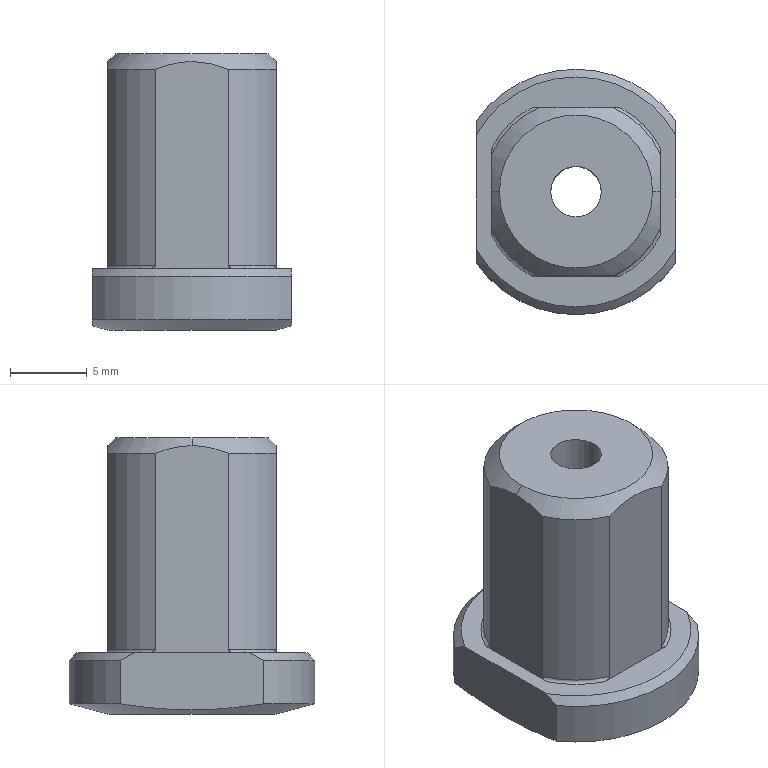Component | SolidWorks | DZ.KX.203-TC1505-30-09-01-05-18-1 | 1 solid | 27 faces | box 13 x 16 x 18 mm | volume 2023 mm3 | plane 9 | cylinder 8 | cone 6 | torus 4 | commonest cylinder face diameters 12 x4 3.3 x2 16 x2
STEP:
#1=COLOUR_RGB('',0.7922,0.8196,0.9333);
#2=FILL_AREA_STYLE_COLOUR('',#1);
#3=FILL_AREA_STYLE('',(#2));
#4=SURFACE_STYLE_FILL_AREA(#3);
#5=SURFACE_SIDE_STYLE('',(#4));
#6=SURFACE_STYLE_USAGE(.BOTH.,#5);
#7=PRESENTATION_STYLE_ASSIGNMENT((#6));
#8=CARTESIAN_POINT('',(11.53,-22.689,0.6716));
#9=VERTEX_POINT('',#8);
#10=CARTESIAN_POINT('',(11.659,-22.689,0.6716));
#11=VERTEX_POINT('',#10);
#12=CARTESIAN_POINT('',(11.594,-22.689,0.6716));
#13=DIRECTION('',(0.,0.,1.));
#14=DIRECTION('',(1.,0.,0.));
#15=AXIS2_PLACEMENT_3D('',#12,#13,#14);
#16=CIRCLE('',#15,0.06496);
#17=EDGE_CURVE('',#9,#11,#16,.T.);
#18=ORIENTED_EDGE('',*,*,#17,.F.);
#19=CARTESIAN_POINT('',(11.53,-22.689,1.38));
#20=VERTEX_POINT('',#19);
#21=CARTESIAN_POINT('',(11.53,-22.689,1.38));
#22=DIRECTION('',(0.,0.,1.));
#23=VECTOR('',#22,39.37);
#24=LINE('',#21,#23);
#25=EDGE_CURVE('',#9,#20,#24,.T.);
#26=ORIENTED_EDGE('',*,*,#25,.T.);
#27=CARTESIAN_POINT('',(11.659,-22.689,1.38));
#28=VERTEX_POINT('',#27);
#29=CARTESIAN_POINT('',(11.594,-22.689,1.38));
#30=DIRECTION('',(0.,0.,1.));
#31=DIRECTION('',(1.,0.,0.));
#32=AXIS2_PLACEMENT_3D('',#29,#30,#31);
#33=CIRCLE('',#32,0.06496);
#34=EDGE_CURVE('',#20,#28,#33,.T.);
#35=ORIENTED_EDGE('',*,*,#34,.T.);
#36=CARTESIAN_POINT('',(11.659,-22.689,1.38));
#37=DIRECTION('',(0.,0.,1.));
#38=VECTOR('',#37,39.37);
#39=LINE('',#36,#38);
#40=EDGE_CURVE('',#11,#28,#39,.T.);
#41=ORIENTED_EDGE('',*,*,#40,.F.);
#42=EDGE_LOOP('',(#18,#26,#35,#41));
#43=FACE_OUTER_BOUND('',#42,.T.);
#44=CARTESIAN_POINT('',(11.594,-22.689,1.38));
#45=DIRECTION('',(0.,0.,1.));
#46=DIRECTION('',(1.,0.,0.));
#47=AXIS2_PLACEMENT_3D('',#44,#45,#46);
#48=CYLINDRICAL_SURFACE('',#47,0.06496);
#49=ADVANCED_FACE('',(#43),#48,.F.);
#50=CARTESIAN_POINT('',(11.378,-22.689,0.6716));
#51=VERTEX_POINT('',#50);
#52=CARTESIAN_POINT('',(11.811,-22.689,0.6716));
#53=VERTEX_POINT('',#52);
#54=CARTESIAN_POINT('',(11.594,-22.689,0.6716));
#55=DIRECTION('',(-0.,-0.,-1.));
#56=DIRECTION('',(-1.,0.,0.));
#57=AXIS2_PLACEMENT_3D('',#54,#55,#56);
#58=CIRCLE('',#57,0.2165);
#59=EDGE_CURVE('',#51,#53,#58,.T.);
#60=ORIENTED_EDGE('',*,*,#59,.F.);
#61=CARTESIAN_POINT('',(11.339,-22.689,0.6822));
#62=VERTEX_POINT('',#61);
#63=CARTESIAN_POINT('',(11.28,-22.689,0.698));
#64=DIRECTION('',(-0.9659,0.,0.2588));
#65=VECTOR('',#64,39.37);
#66=LINE('',#63,#65);
#67=EDGE_CURVE('',#51,#62,#66,.T.);
#68=ORIENTED_EDGE('',*,*,#67,.T.);
#69=CARTESIAN_POINT('',(11.339,-22.506,0.698));
#70=VERTEX_POINT('',#69);
#71=CARTESIAN_POINT('',(11.339,-22.689,0.6822));
#72=CARTESIAN_POINT('',(11.339,-22.659,0.6822));
#73=CARTESIAN_POINT('',(11.339,-22.628,0.6837));
#74=CARTESIAN_POINT('',(11.339,-22.567,0.6892));
#75=CARTESIAN_POINT('',(11.339,-22.536,0.6933));
#76=CARTESIAN_POINT('',(11.339,-22.506,0.698));
#77=B_SPLINE_CURVE_WITH_KNOTS('',3,(#71,#72,#73,#74,#75,#76),.UNSPECIFIED.,.F.,.F.,(4,2,4),(0.0133,0.01565,0.018),.UNSPECIFIED.);
#78=EDGE_CURVE('',#62,#70,#77,.T.);
#79=ORIENTED_EDGE('',*,*,#78,.T.);
#80=CARTESIAN_POINT('',(11.85,-22.506,0.698));
#81=VERTEX_POINT('',#80);
#82=CARTESIAN_POINT('',(11.594,-22.689,0.698));
#83=DIRECTION('',(-0.,-0.,-1.));
#84=DIRECTION('',(-1.,0.,0.));
#85=AXIS2_PLACEMENT_3D('',#82,#83,#84);
#86=CIRCLE('',#85,0.315);
#87=EDGE_CURVE('',#70,#81,#86,.T.);
#88=ORIENTED_EDGE('',*,*,#87,.T.);
#89=CARTESIAN_POINT('',(11.85,-22.689,0.6822));
#90=VERTEX_POINT('',#89);
#91=CARTESIAN_POINT('',(11.85,-22.506,0.698));
#92=CARTESIAN_POINT('',(11.85,-22.536,0.6933));
#93=CARTESIAN_POINT('',(11.85,-22.567,0.6892));
#94=CARTESIAN_POINT('',(11.85,-22.628,0.6837));
#95=CARTESIAN_POINT('',(11.85,-22.659,0.6822));
#96=CARTESIAN_POINT('',(11.85,-22.689,0.6822));
#97=B_SPLINE_CURVE_WITH_KNOTS('',3,(#91,#92,#93,#94,#95,#96),.UNSPECIFIED.,.F.,.F.,(4,2,4),(0.02781,0.03015,0.03249),.UNSPECIFIED.);
#98=EDGE_CURVE('',#81,#90,#97,.T.);
#99=ORIENTED_EDGE('',*,*,#98,.T.);
#100=CARTESIAN_POINT('',(11.909,-22.689,0.698));
#101=DIRECTION('',(0.9659,0.,0.2588));
#102=VECTOR('',#101,39.37);
#103=LINE('',#100,#102);
#104=EDGE_CURVE('',#53,#90,#103,.T.);
#105=ORIENTED_EDGE('',*,*,#104,.F.);
#106=EDGE_LOOP('',(#60,#68,#79,#88,#99,#105));
#107=FACE_OUTER_BOUND('',#106,.T.);
#108=CARTESIAN_POINT('',(11.594,-22.689,0.698));
#109=DIRECTION('',(0.,0.,1.));
#110=DIRECTION('',(1.,0.,-0.));
#111=AXIS2_PLACEMENT_3D('',#108,#109,#110);
#112=CONICAL_SURFACE('',#111,0.315,1.309);
#113=ADVANCED_FACE('',(#107),#112,.T.);
#114=CARTESIAN_POINT('',(11.398,-22.689,1.38));
#115=VERTEX_POINT('',#114);
#116=CARTESIAN_POINT('',(11.791,-22.689,1.38));
#117=VERTEX_POINT('',#116);
#118=CARTESIAN_POINT('',(11.594,-22.689,1.38));
#119=DIRECTION('',(-0.,-0.,-1.));
#120=DIRECTION('',(-1.,0.,0.));
#121=AXIS2_PLACEMENT_3D('',#118,#119,#120);
#122=CIRCLE('',#121,0.1969);
#123=EDGE_CURVE('',#115,#117,#122,.T.);
#124=ORIENTED_EDGE('',*,*,#123,.T.);
#125=CARTESIAN_POINT('',(11.811,-22.689,1.361));
#126=VERTEX_POINT('',#125);
#127=CARTESIAN_POINT('',(11.791,-22.689,1.38));
#128=DIRECTION('',(0.7071,-0.,-0.7071));
#129=VECTOR('',#128,39.37);
#130=LINE('',#127,#129);
#131=EDGE_CURVE('',#117,#126,#130,.T.);
#132=ORIENTED_EDGE('',*,*,#131,.T.);
#133=CARTESIAN_POINT('',(11.811,-22.595,1.341));
#134=VERTEX_POINT('',#133);
#135=CARTESIAN_POINT('',(11.811,-22.595,1.341));
#136=CARTESIAN_POINT('',(11.811,-22.61,1.347));
#137=CARTESIAN_POINT('',(11.811,-22.625,1.352));
#138=CARTESIAN_POINT('',(11.811,-22.649,1.357));
#139=CARTESIAN_POINT('',(11.811,-22.657,1.358));
#140=CARTESIAN_POINT('',(11.811,-22.673,1.36));
#141=CARTESIAN_POINT('',(11.811,-22.681,1.361));
#142=CARTESIAN_POINT('',(11.811,-22.689,1.361));
#143=B_SPLINE_CURVE_WITH_KNOTS('',3,(#135,#136,#137,#138,#139,#140,#141,#142),.UNSPECIFIED.,.F.,.F.,(4,2,2,4),(0.004827,0.006044,0.006653,0.007262),.UNSPECIFIED.);
#144=EDGE_CURVE('',#134,#126,#143,.T.);
#145=ORIENTED_EDGE('',*,*,#144,.F.);
#146=CARTESIAN_POINT('',(11.689,-22.473,1.341));
#147=VERTEX_POINT('',#146);
#148=CARTESIAN_POINT('',(11.594,-22.689,1.341));
#149=DIRECTION('',(-0.,-0.,-1.));
#150=DIRECTION('',(-1.,0.,0.));
#151=AXIS2_PLACEMENT_3D('',#148,#149,#150);
#152=CIRCLE('',#151,0.2362);
#153=EDGE_CURVE('',#147,#134,#152,.T.);
#154=ORIENTED_EDGE('',*,*,#153,.F.);
#155=CARTESIAN_POINT('',(11.5,-22.473,1.341));
#156=VERTEX_POINT('',#155);
#157=CARTESIAN_POINT('',(11.5,-22.473,1.341));
#158=CARTESIAN_POINT('',(11.515,-22.473,1.347));
#159=CARTESIAN_POINT('',(11.531,-22.473,1.352));
#160=CARTESIAN_POINT('',(11.554,-22.473,1.357));
#161=CARTESIAN_POINT('',(11.562,-22.473,1.358));
#162=CARTESIAN_POINT('',(11.578,-22.473,1.36));
#163=CARTESIAN_POINT('',(11.587,-22.473,1.361));
#164=CARTESIAN_POINT('',(11.611,-22.473,1.361));
#165=CARTESIAN_POINT('',(11.627,-22.473,1.359));
#166=CARTESIAN_POINT('',(11.659,-22.473,1.352));
#167=CARTESIAN_POINT('',(11.674,-22.473,1.347));
#168=CARTESIAN_POINT('',(11.689,-22.473,1.341));
#169=B_SPLINE_CURVE_WITH_KNOTS('',3,(#157,#158,#159,#160,#161,#162,#163,#164,#165,#166,#167,#168),.UNSPECIFIED.,.F.,.F.,(4,2,2,2,2,4),(0.004827,0.006047,0.006657,0.007266,0.008486,0.009706),.UNSPECIFIED.);
#170=EDGE_CURVE('',#156,#147,#169,.T.);
#171=ORIENTED_EDGE('',*,*,#170,.F.);
#172=CARTESIAN_POINT('',(11.378,-22.595,1.341));
#173=VERTEX_POINT('',#172);
#174=CARTESIAN_POINT('',(11.594,-22.689,1.341));
#175=DIRECTION('',(-0.,-0.,-1.));
#176=DIRECTION('',(-1.,0.,0.));
#177=AXIS2_PLACEMENT_3D('',#174,#175,#176);
#178=CIRCLE('',#177,0.2362);
#179=EDGE_CURVE('',#173,#156,#178,.T.);
#180=ORIENTED_EDGE('',*,*,#179,.F.);
#181=CARTESIAN_POINT('',(11.378,-22.689,1.361));
#182=VERTEX_POINT('',#181);
#183=CARTESIAN_POINT('',(11.378,-22.689,1.361));
#184=CARTESIAN_POINT('',(11.378,-22.681,1.361));
#185=CARTESIAN_POINT('',(11.378,-22.673,1.36));
#186=CARTESIAN_POINT('',(11.378,-22.657,1.358));
#187=CARTESIAN_POINT('',(11.378,-22.649,1.357));
#188=CARTESIAN_POINT('',(11.378,-22.625,1.352));
#189=CARTESIAN_POINT('',(11.378,-22.61,1.347));
#190=CARTESIAN_POINT('',(11.378,-22.595,1.341));
#191=B_SPLINE_CURVE_WITH_KNOTS('',3,(#183,#184,#185,#186,#187,#188,#189,#190),.UNSPECIFIED.,.F.,.F.,(4,2,2,4),(0.01553,0.01614,0.01674,0.01796),.UNSPECIFIED.);
#192=EDGE_CURVE('',#182,#173,#191,.T.);
#193=ORIENTED_EDGE('',*,*,#192,.F.);
#194=CARTESIAN_POINT('',(11.398,-22.689,1.38));
#195=DIRECTION('',(-0.7071,-0.,-0.7071));
#196=VECTOR('',#195,39.37);
#197=LINE('',#194,#196);
#198=EDGE_CURVE('',#115,#182,#197,.T.);
#199=ORIENTED_EDGE('',*,*,#198,.F.);
#200=EDGE_LOOP('',(#124,#132,#145,#154,#171,#180,#193,#199));
#201=FACE_OUTER_BOUND('',#200,.T.);
#202=CARTESIAN_POINT('',(11.594,-22.689,1.38));
#203=DIRECTION('',(-0.,-0.,-1.));
#204=DIRECTION('',(-1.,0.,0.));
#205=AXIS2_PLACEMENT_3D('',#202,#203,#204);
#206=CONICAL_SURFACE('',#205,0.1969,0.7854);
#207=ADVANCED_FACE('',(#201),#206,.T.);
#208=ORIENTED_EDGE('',*,*,#131,.F.);
#209=CARTESIAN_POINT('',(11.594,-22.689,1.38));
#210=DIRECTION('',(-0.,-0.,-1.));
#211=DIRECTION('',(-1.,0.,0.));
#212=AXIS2_PLACEMENT_3D('',#209,#210,#211);
#213=CIRCLE('',#212,0.1969);
#214=EDGE_CURVE('',#117,#115,#213,.T.);
#215=ORIENTED_EDGE('',*,*,#214,.T.);
#216=ORIENTED_EDGE('',*,*,#198,.T.);
#217=CARTESIAN_POINT('',(11.378,-22.784,1.341));
#218=VERTEX_POINT('',#217);
#219=CARTESIAN_POINT('',(11.378,-22.784,1.341));
#220=CARTESIAN_POINT('',(11.378,-22.769,1.347));
#221=CARTESIAN_POINT('',(11.378,-22.753,1.352));
#222=CARTESIAN_POINT('',(11.378,-22.722,1.359));
#223=CARTESIAN_POINT('',(11.378,-22.705,1.361));
#224=CARTESIAN_POINT('',(11.378,-22.689,1.361));
#225=B_SPLINE_CURVE_WITH_KNOTS('',3,(#219,#220,#221,#222,#223,#224),.UNSPECIFIED.,.F.,.F.,(4,2,4),(0.01309,0.01431,0.01553),.UNSPECIFIED.);
#226=EDGE_CURVE('',#218,#182,#225,.T.);
#227=ORIENTED_EDGE('',*,*,#226,.F.);
#228=CARTESIAN_POINT('',(11.5,-22.906,1.341));
#229=VERTEX_POINT('',#228);
#230=CARTESIAN_POINT('',(11.594,-22.689,1.341));
#231=DIRECTION('',(-0.,-0.,-1.));
#232=DIRECTION('',(-1.,0.,0.));
#233=AXIS2_PLACEMENT_3D('',#230,#231,#232);
#234=CIRCLE('',#233,0.2362);
#235=EDGE_CURVE('',#229,#218,#234,.T.);
#236=ORIENTED_EDGE('',*,*,#235,.F.);
#237=CARTESIAN_POINT('',(11.689,-22.906,1.341));
#238=VERTEX_POINT('',#237);
#239=CARTESIAN_POINT('',(11.689,-22.906,1.341));
#240=CARTESIAN_POINT('',(11.674,-22.906,1.347));
#241=CARTESIAN_POINT('',(11.659,-22.906,1.352));
#242=CARTESIAN_POINT('',(11.627,-22.906,1.359));
#243=CARTESIAN_POINT('',(11.611,-22.906,1.361));
#244=CARTESIAN_POINT('',(11.587,-22.906,1.361));
#245=CARTESIAN_POINT('',(11.578,-22.906,1.36));
#246=CARTESIAN_POINT('',(11.562,-22.906,1.358));
#247=CARTESIAN_POINT('',(11.554,-22.906,1.357));
#248=CARTESIAN_POINT('',(11.531,-22.906,1.352));
#249=CARTESIAN_POINT('',(11.515,-22.906,1.347));
#250=CARTESIAN_POINT('',(11.5,-22.906,1.341));
#251=B_SPLINE_CURVE_WITH_KNOTS('',3,(#239,#240,#241,#242,#243,#244,#245,#246,#247,#248,#249,#250),.UNSPECIFIED.,.F.,.F.,(4,2,2,2,2,4),(0.01309,0.01431,0.01553,0.01613,0.01674,0.01796),.UNSPECIFIED.);
#252=EDGE_CURVE('',#238,#229,#251,.T.);
#253=ORIENTED_EDGE('',*,*,#252,.F.);
#254=CARTESIAN_POINT('',(11.811,-22.784,1.341));
#255=VERTEX_POINT('',#254);
#256=CARTESIAN_POINT('',(11.594,-22.689,1.341));
#257=DIRECTION('',(-0.,-0.,-1.));
#258=DIRECTION('',(-1.,0.,0.));
#259=AXIS2_PLACEMENT_3D('',#256,#257,#258);
#260=CIRCLE('',#259,0.2362);
#261=EDGE_CURVE('',#255,#238,#260,.T.);
#262=ORIENTED_EDGE('',*,*,#261,.F.);
#263=CARTESIAN_POINT('',(11.811,-22.689,1.361));
#264=CARTESIAN_POINT('',(11.811,-22.705,1.361));
#265=CARTESIAN_POINT('',(11.811,-22.722,1.359));
#266=CARTESIAN_POINT('',(11.811,-22.753,1.352));
#267=CARTESIAN_POINT('',(11.811,-22.769,1.347));
#268=CARTESIAN_POINT('',(11.811,-22.784,1.341));
#269=B_SPLINE_CURVE_WITH_KNOTS('',3,(#263,#264,#265,#266,#267,#268),.UNSPECIFIED.,.F.,.F.,(4,2,4),(0.007262,0.008484,0.009706),.UNSPECIFIED.);
#270=EDGE_CURVE('',#126,#255,#269,.T.);
#271=ORIENTED_EDGE('',*,*,#270,.F.);
#272=EDGE_LOOP('',(#208,#215,#216,#227,#236,#253,#262,#271));
#273=FACE_OUTER_BOUND('',#272,.T.);
#274=CARTESIAN_POINT('',(11.594,-22.689,1.38));
#275=DIRECTION('',(-0.,-0.,-1.));
#276=DIRECTION('',(-1.,0.,0.));
#277=AXIS2_PLACEMENT_3D('',#274,#275,#276);
#278=CONICAL_SURFACE('',#277,0.1969,0.7854);
#279=ADVANCED_FACE('',(#273),#278,.T.);
#280=CARTESIAN_POINT('',(11.811,-22.784,0.837));
#281=VERTEX_POINT('',#280);
#282=CARTESIAN_POINT('',(11.811,-22.784,1.065));
#283=DIRECTION('',(-0.,-0.,-1.));
#284=VECTOR('',#283,39.37);
#285=LINE('',#282,#284);
#286=EDGE_CURVE('',#255,#281,#285,.T.);
#287=ORIENTED_EDGE('',*,*,#286,.F.);
#288=ORIENTED_EDGE('',*,*,#261,.T.);
#289=CARTESIAN_POINT('',(11.689,-22.906,0.837));
#290=VERTEX_POINT('',#289);
#291=CARTESIAN_POINT('',(11.689,-22.906,1.065));
#292=DIRECTION('',(0.,0.,1.));
#293=VECTOR('',#292,39.37);
#294=LINE('',#291,#293);
#295=EDGE_CURVE('',#290,#238,#294,.T.);
#296=ORIENTED_EDGE('',*,*,#295,.F.);
#297=CARTESIAN_POINT('',(11.594,-22.689,0.837));
#298=DIRECTION('',(-0.,-0.,-1.));
#299=DIRECTION('',(-1.,0.,0.));
#300=AXIS2_PLACEMENT_3D('',#297,#298,#299);
#301=CIRCLE('',#300,0.2362);
#302=EDGE_CURVE('',#281,#290,#301,.T.);
#303=ORIENTED_EDGE('',*,*,#302,.F.);
#304=EDGE_LOOP('',(#287,#288,#296,#303));
#305=FACE_OUTER_BOUND('',#304,.T.);
#306=CARTESIAN_POINT('',(11.594,-22.689,1.065));
#307=DIRECTION('',(-0.,-0.,-1.));
#308=DIRECTION('',(-1.,0.,0.));
#309=AXIS2_PLACEMENT_3D('',#306,#307,#308);
#310=CYLINDRICAL_SURFACE('',#309,0.2362);
#311=ADVANCED_FACE('',(#305),#310,.T.);
#312=CARTESIAN_POINT('',(11.811,-22.595,0.837));
#313=VERTEX_POINT('',#312);
#314=CARTESIAN_POINT('',(11.811,-22.595,1.065));
#315=DIRECTION('',(0.,0.,1.));
#316=VECTOR('',#315,39.37);
#317=LINE('',#314,#316);
#318=EDGE_CURVE('',#313,#134,#317,.T.);
#319=ORIENTED_EDGE('',*,*,#318,.F.);
#320=CARTESIAN_POINT('',(11.689,-22.473,0.837));
#321=VERTEX_POINT('',#320);
#322=CARTESIAN_POINT('',(11.594,-22.689,0.837));
#323=DIRECTION('',(-0.,-0.,-1.));
#324=DIRECTION('',(-1.,0.,0.));
#325=AXIS2_PLACEMENT_3D('',#322,#323,#324);
#326=CIRCLE('',#325,0.2362);
#327=EDGE_CURVE('',#321,#313,#326,.T.);
#328=ORIENTED_EDGE('',*,*,#327,.F.);
#329=CARTESIAN_POINT('',(11.689,-22.473,1.065));
#330=DIRECTION('',(-0.,-0.,-1.));
#331=VECTOR('',#330,39.37);
#332=LINE('',#329,#331);
#333=EDGE_CURVE('',#147,#321,#332,.T.);
#334=ORIENTED_EDGE('',*,*,#333,.F.);
#335=ORIENTED_EDGE('',*,*,#153,.T.);
#336=EDGE_LOOP('',(#319,#328,#334,#335));
#337=FACE_OUTER_BOUND('',#336,.T.);
#338=CARTESIAN_POINT('',(11.594,-22.689,1.065));
#339=DIRECTION('',(-0.,-0.,-1.));
#340=DIRECTION('',(-1.,0.,0.));
#341=AXIS2_PLACEMENT_3D('',#338,#339,#340);
#342=CYLINDRICAL_SURFACE('',#341,0.2362);
#343=ADVANCED_FACE('',(#337),#342,.T.);
#344=CARTESIAN_POINT('',(11.5,-22.906,0.837));
#345=VERTEX_POINT('',#344);
#346=CARTESIAN_POINT('',(11.5,-22.906,1.065));
#347=DIRECTION('',(-0.,-0.,-1.));
#348=VECTOR('',#347,39.37);
#349=LINE('',#346,#348);
#350=EDGE_CURVE('',#229,#345,#349,.T.);
#351=ORIENTED_EDGE('',*,*,#350,.F.);
#352=ORIENTED_EDGE('',*,*,#235,.T.);
#353=CARTESIAN_POINT('',(11.378,-22.784,0.837));
#354=VERTEX_POINT('',#353);
#355=CARTESIAN_POINT('',(11.378,-22.784,1.065));
#356=DIRECTION('',(0.,0.,1.));
#357=VECTOR('',#356,39.37);
#358=LINE('',#355,#357);
#359=EDGE_CURVE('',#354,#218,#358,.T.);
#360=ORIENTED_EDGE('',*,*,#359,.F.);
#361=CARTESIAN_POINT('',(11.594,-22.689,0.837));
#362=DIRECTION('',(-0.,-0.,-1.));
#363=DIRECTION('',(-1.,0.,0.));
#364=AXIS2_PLACEMENT_3D('',#361,#362,#363);
#365=CIRCLE('',#364,0.2362);
#366=EDGE_CURVE('',#345,#354,#365,.T.);
#367=ORIENTED_EDGE('',*,*,#366,.F.);
#368=EDGE_LOOP('',(#351,#352,#360,#367));
#369=FACE_OUTER_BOUND('',#368,.T.);
#370=CARTESIAN_POINT('',(11.594,-22.689,1.065));
#371=DIRECTION('',(-0.,-0.,-1.));
#372=DIRECTION('',(-1.,0.,0.));
#373=AXIS2_PLACEMENT_3D('',#370,#371,#372);
#374=CYLINDRICAL_SURFACE('',#373,0.2362);
#375=ADVANCED_FACE('',(#369),#374,.T.);
#376=CARTESIAN_POINT('',(11.378,-22.595,0.837));
#377=VERTEX_POINT('',#376);
#378=CARTESIAN_POINT('',(11.378,-22.595,1.065));
#379=DIRECTION('',(-0.,-0.,-1.));
#380=VECTOR('',#379,39.37);
#381=LINE('',#378,#380);
#382=EDGE_CURVE('',#173,#377,#381,.T.);
#383=ORIENTED_EDGE('',*,*,#382,.F.);
#384=ORIENTED_EDGE('',*,*,#179,.T.);
#385=CARTESIAN_POINT('',(11.5,-22.473,0.837));
#386=VERTEX_POINT('',#385);
#387=CARTESIAN_POINT('',(11.5,-22.473,1.065));
#388=DIRECTION('',(0.,0.,1.));
#389=VECTOR('',#388,39.37);
#390=LINE('',#387,#389);
#391=EDGE_CURVE('',#386,#156,#390,.T.);
#392=ORIENTED_EDGE('',*,*,#391,.F.);
#393=CARTESIAN_POINT('',(11.594,-22.689,0.837));
#394=DIRECTION('',(-0.,-0.,-1.));
#395=DIRECTION('',(-1.,0.,0.));
#396=AXIS2_PLACEMENT_3D('',#393,#394,#395);
#397=CIRCLE('',#396,0.2362);
#398=EDGE_CURVE('',#377,#386,#397,.T.);
#399=ORIENTED_EDGE('',*,*,#398,.F.);
#400=EDGE_LOOP('',(#383,#384,#392,#399));
#401=FACE_OUTER_BOUND('',#400,.T.);
#402=CARTESIAN_POINT('',(11.594,-22.689,1.065));
#403=DIRECTION('',(-0.,-0.,-1.));
#404=DIRECTION('',(-1.,0.,0.));
#405=AXIS2_PLACEMENT_3D('',#402,#403,#404);
#406=CYLINDRICAL_SURFACE('',#405,0.2362);
#407=ADVANCED_FACE('',(#401),#406,.T.);
#408=CARTESIAN_POINT('',(11.811,-22.802,0.8291));
#409=VERTEX_POINT('',#408);
#410=CARTESIAN_POINT('',(11.811,-22.784,0.837));
#411=CARTESIAN_POINT('',(11.811,-22.784,0.8361));
#412=CARTESIAN_POINT('',(11.811,-22.784,0.8352));
#413=CARTESIAN_POINT('',(11.811,-22.785,0.8338));
#414=CARTESIAN_POINT('',(11.811,-22.786,0.8333));
#415=CARTESIAN_POINT('',(11.811,-22.788,0.8318));
#416=CARTESIAN_POINT('',(11.811,-22.79,0.8312));
#417=CARTESIAN_POINT('',(11.811,-22.795,0.8296));
#418=CARTESIAN_POINT('',(11.811,-22.798,0.8291));
#419=CARTESIAN_POINT('',(11.811,-22.802,0.8291));
#420=B_SPLINE_CURVE_WITH_KNOTS('',3,(#410,#411,#412,#413,#414,#415,#416,#417,#418,#419),.UNSPECIFIED.,.F.,.F.,(4,2,2,2,4),(0.001122,0.00119,0.001258,0.001394,0.001665),.UNSPECIFIED.);
#421=EDGE_CURVE('',#281,#409,#420,.T.);
#422=ORIENTED_EDGE('',*,*,#421,.F.);
#423=ORIENTED_EDGE('',*,*,#302,.T.);
#424=CARTESIAN_POINT('',(11.707,-22.906,0.8291));
#425=VERTEX_POINT('',#424);
#426=CARTESIAN_POINT('',(11.707,-22.906,0.8291));
#427=CARTESIAN_POINT('',(11.704,-22.906,0.8291));
#428=CARTESIAN_POINT('',(11.7,-22.906,0.8296));
#429=CARTESIAN_POINT('',(11.695,-22.906,0.8311));
#430=CARTESIAN_POINT('',(11.693,-22.906,0.8318));
#431=CARTESIAN_POINT('',(11.691,-22.906,0.8333));
#432=CARTESIAN_POINT('',(11.69,-22.906,0.8338));
#433=CARTESIAN_POINT('',(11.689,-22.906,0.8352));
#434=CARTESIAN_POINT('',(11.689,-22.906,0.8361));
#435=CARTESIAN_POINT('',(11.689,-22.906,0.837));
#436=B_SPLINE_CURVE_WITH_KNOTS('',3,(#426,#427,#428,#429,#430,#431,#432,#433,#434,#435),.UNSPECIFIED.,.F.,.F.,(4,2,2,2,4),(0.0004163,0.0006859,0.0008207,0.0008881,0.0009555),.UNSPECIFIED.);
#437=EDGE_CURVE('',#425,#290,#436,.T.);
#438=ORIENTED_EDGE('',*,*,#437,.F.);
#439=CARTESIAN_POINT('',(11.594,-22.689,0.8291));
#440=DIRECTION('',(-0.,-0.,-1.));
#441=DIRECTION('',(-1.,0.,0.));
#442=AXIS2_PLACEMENT_3D('',#439,#440,#441);
#443=CIRCLE('',#442,0.2441);
#444=EDGE_CURVE('',#409,#425,#443,.T.);
#445=ORIENTED_EDGE('',*,*,#444,.F.);
#446=EDGE_LOOP('',(#422,#423,#438,#445));
#447=FACE_OUTER_BOUND('',#446,.T.);
#448=CARTESIAN_POINT('',(11.594,-22.689,0.837));
#449=DIRECTION('',(-0.,-0.,-1.));
#450=DIRECTION('',(-1.,-0.,0.));
#451=AXIS2_PLACEMENT_3D('',#448,#449,#450);
#452=TOROIDAL_SURFACE('',#451,0.2441,0.007874);
#453=ADVANCED_FACE('',(#447),#452,.F.);
#454=CARTESIAN_POINT('',(11.811,-22.577,0.8291));
#455=VERTEX_POINT('',#454);
#456=CARTESIAN_POINT('',(11.811,-22.577,0.8291));
#457=CARTESIAN_POINT('',(11.811,-22.58,0.8291));
#458=CARTESIAN_POINT('',(11.811,-22.584,0.8296));
#459=CARTESIAN_POINT('',(11.811,-22.589,0.8311));
#460=CARTESIAN_POINT('',(11.811,-22.59,0.8318));
#461=CARTESIAN_POINT('',(11.811,-22.593,0.8333));
#462=CARTESIAN_POINT('',(11.811,-22.593,0.8338));
#463=CARTESIAN_POINT('',(11.811,-22.594,0.8352));
#464=CARTESIAN_POINT('',(11.811,-22.595,0.8361));
#465=CARTESIAN_POINT('',(11.811,-22.595,0.837));
#466=B_SPLINE_CURVE_WITH_KNOTS('',3,(#456,#457,#458,#459,#460,#461,#462,#463,#464,#465),.UNSPECIFIED.,.F.,.F.,(4,2,2,2,4),(0.001507,0.001778,0.001913,0.001981,0.002048),.UNSPECIFIED.);
#467=EDGE_CURVE('',#455,#313,#466,.T.);
#468=ORIENTED_EDGE('',*,*,#467,.F.);
#469=CARTESIAN_POINT('',(11.707,-22.473,0.8291));
#470=VERTEX_POINT('',#469);
#471=CARTESIAN_POINT('',(11.594,-22.689,0.8291));
#472=DIRECTION('',(-0.,-0.,-1.));
#473=DIRECTION('',(-1.,0.,0.));
#474=AXIS2_PLACEMENT_3D('',#471,#472,#473);
#475=CIRCLE('',#474,0.2441);
#476=EDGE_CURVE('',#470,#455,#475,.T.);
#477=ORIENTED_EDGE('',*,*,#476,.F.);
#478=CARTESIAN_POINT('',(11.689,-22.473,0.837));
#479=CARTESIAN_POINT('',(11.689,-22.473,0.8361));
#480=CARTESIAN_POINT('',(11.689,-22.473,0.8352));
#481=CARTESIAN_POINT('',(11.69,-22.473,0.8338));
#482=CARTESIAN_POINT('',(11.691,-22.473,0.8333));
#483=CARTESIAN_POINT('',(11.693,-22.473,0.8318));
#484=CARTESIAN_POINT('',(11.695,-22.473,0.8312));
#485=CARTESIAN_POINT('',(11.7,-22.473,0.8296));
#486=CARTESIAN_POINT('',(11.704,-22.473,0.8291));
#487=CARTESIAN_POINT('',(11.707,-22.473,0.8291));
#488=B_SPLINE_CURVE_WITH_KNOTS('',3,(#478,#479,#480,#481,#482,#483,#484,#485,#486,#487),.UNSPECIFIED.,.F.,.F.,(4,2,2,2,4),(0.001122,0.00119,0.001258,0.001394,0.001665),.UNSPECIFIED.);
#489=EDGE_CURVE('',#321,#470,#488,.T.);
#490=ORIENTED_EDGE('',*,*,#489,.F.);
#491=ORIENTED_EDGE('',*,*,#327,.T.);
#492=EDGE_LOOP('',(#468,#477,#490,#491));
#493=FACE_OUTER_BOUND('',#492,.T.);
#494=CARTESIAN_POINT('',(11.594,-22.689,0.837));
#495=DIRECTION('',(-0.,-0.,-1.));
#496=DIRECTION('',(-1.,-0.,0.));
#497=AXIS2_PLACEMENT_3D('',#494,#495,#496);
#498=TOROIDAL_SURFACE('',#497,0.2441,0.007874);
#499=ADVANCED_FACE('',(#493),#498,.F.);
#500=CARTESIAN_POINT('',(11.482,-22.906,0.8291));
#501=VERTEX_POINT('',#500);
#502=CARTESIAN_POINT('',(11.5,-22.906,0.837));
#503=CARTESIAN_POINT('',(11.5,-22.906,0.8361));
#504=CARTESIAN_POINT('',(11.5,-22.906,0.8352));
#505=CARTESIAN_POINT('',(11.499,-22.906,0.8338));
#506=CARTESIAN_POINT('',(11.498,-22.906,0.8333));
#507=CARTESIAN_POINT('',(11.496,-22.906,0.8318));
#508=CARTESIAN_POINT('',(11.494,-22.906,0.8312));
#509=CARTESIAN_POINT('',(11.489,-22.906,0.8296));
#510=CARTESIAN_POINT('',(11.485,-22.906,0.8291));
#511=CARTESIAN_POINT('',(11.482,-22.906,0.8291));
#512=B_SPLINE_CURVE_WITH_KNOTS('',3,(#502,#503,#504,#505,#506,#507,#508,#509,#510,#511),.UNSPECIFIED.,.F.,.F.,(4,2,2,2,4),(0.00002678,0.00009477,0.0001628,0.0002987,0.0005707),.UNSPECIFIED.);
#513=EDGE_CURVE('',#345,#501,#512,.T.);
#514=ORIENTED_EDGE('',*,*,#513,.F.);
#515=ORIENTED_EDGE('',*,*,#366,.T.);
#516=CARTESIAN_POINT('',(11.378,-22.802,0.8291));
#517=VERTEX_POINT('',#516);
#518=CARTESIAN_POINT('',(11.378,-22.802,0.8291));
#519=CARTESIAN_POINT('',(11.378,-22.798,0.8291));
#520=CARTESIAN_POINT('',(11.378,-22.795,0.8296));
#521=CARTESIAN_POINT('',(11.378,-22.79,0.8311));
#522=CARTESIAN_POINT('',(11.378,-22.788,0.8318));
#523=CARTESIAN_POINT('',(11.378,-22.786,0.8333));
#524=CARTESIAN_POINT('',(11.378,-22.785,0.8338));
#525=CARTESIAN_POINT('',(11.378,-22.784,0.8352));
#526=CARTESIAN_POINT('',(11.378,-22.784,0.8361));
#527=CARTESIAN_POINT('',(11.378,-22.784,0.837));
#528=B_SPLINE_CURVE_WITH_KNOTS('',3,(#518,#519,#520,#521,#522,#523,#524,#525,#526,#527),.UNSPECIFIED.,.F.,.F.,(4,2,2,2,4),(0.0004163,0.0006859,0.0008207,0.0008881,0.0009555),.UNSPECIFIED.);
#529=EDGE_CURVE('',#517,#354,#528,.T.);
#530=ORIENTED_EDGE('',*,*,#529,.F.);
#531=CARTESIAN_POINT('',(11.594,-22.689,0.8291));
#532=DIRECTION('',(-0.,-0.,-1.));
#533=DIRECTION('',(-1.,0.,0.));
#534=AXIS2_PLACEMENT_3D('',#531,#532,#533);
#535=CIRCLE('',#534,0.2441);
#536=EDGE_CURVE('',#501,#517,#535,.T.);
#537=ORIENTED_EDGE('',*,*,#536,.F.);
#538=EDGE_LOOP('',(#514,#515,#530,#537));
#539=FACE_OUTER_BOUND('',#538,.T.);
#540=CARTESIAN_POINT('',(11.594,-22.689,0.837));
#541=DIRECTION('',(-0.,-0.,-1.));
#542=DIRECTION('',(-1.,-0.,0.));
#543=AXIS2_PLACEMENT_3D('',#540,#541,#542);
#544=TOROIDAL_SURFACE('',#543,0.2441,0.007874);
#545=ADVANCED_FACE('',(#539),#544,.F.);
#546=CARTESIAN_POINT('',(11.378,-22.577,0.8291));
#547=VERTEX_POINT('',#546);
#548=CARTESIAN_POINT('',(11.378,-22.595,0.837));
#549=CARTESIAN_POINT('',(11.378,-22.595,0.8361));
#550=CARTESIAN_POINT('',(11.378,-22.594,0.8352));
#551=CARTESIAN_POINT('',(11.378,-22.593,0.8338));
#552=CARTESIAN_POINT('',(11.378,-22.593,0.8333));
#553=CARTESIAN_POINT('',(11.378,-22.59,0.8318));
#554=CARTESIAN_POINT('',(11.378,-22.589,0.8312));
#555=CARTESIAN_POINT('',(11.378,-22.584,0.8296));
#556=CARTESIAN_POINT('',(11.378,-22.58,0.8291));
#557=CARTESIAN_POINT('',(11.378,-22.577,0.8291));
#558=B_SPLINE_CURVE_WITH_KNOTS('',3,(#548,#549,#550,#551,#552,#553,#554,#555,#556,#557),.UNSPECIFIED.,.F.,.F.,(4,2,2,2,4),(0.00002678,0.00009477,0.0001628,0.0002987,0.0005707),.UNSPECIFIED.);
#559=EDGE_CURVE('',#377,#547,#558,.T.);
#560=ORIENTED_EDGE('',*,*,#559,.F.);
#561=ORIENTED_EDGE('',*,*,#398,.T.);
#562=CARTESIAN_POINT('',(11.482,-22.473,0.8291));
#563=VERTEX_POINT('',#562);
#564=CARTESIAN_POINT('',(11.482,-22.473,0.8291));
#565=CARTESIAN_POINT('',(11.485,-22.473,0.8291));
#566=CARTESIAN_POINT('',(11.489,-22.473,0.8296));
#567=CARTESIAN_POINT('',(11.494,-22.473,0.8311));
#568=CARTESIAN_POINT('',(11.496,-22.473,0.8318));
#569=CARTESIAN_POINT('',(11.498,-22.473,0.8333));
#570=CARTESIAN_POINT('',(11.499,-22.473,0.8338));
#571=CARTESIAN_POINT('',(11.5,-22.473,0.8352));
#572=CARTESIAN_POINT('',(11.5,-22.473,0.8361));
#573=CARTESIAN_POINT('',(11.5,-22.473,0.837));
#574=B_SPLINE_CURVE_WITH_KNOTS('',3,(#564,#565,#566,#567,#568,#569,#570,#571,#572,#573),.UNSPECIFIED.,.F.,.F.,(4,2,2,2,4),(0.001507,0.001778,0.001913,0.001981,0.002048),.UNSPECIFIED.);
#575=EDGE_CURVE('',#563,#386,#574,.T.);
#576=ORIENTED_EDGE('',*,*,#575,.F.);
#577=CARTESIAN_POINT('',(11.594,-22.689,0.8291));
#578=DIRECTION('',(-0.,-0.,-1.));
#579=DIRECTION('',(-1.,0.,0.));
#580=AXIS2_PLACEMENT_3D('',#577,#578,#579);
#581=CIRCLE('',#580,0.2441);
#582=EDGE_CURVE('',#547,#563,#581,.T.);
#583=ORIENTED_EDGE('',*,*,#582,.F.);
#584=EDGE_LOOP('',(#560,#561,#576,#583));
#585=FACE_OUTER_BOUND('',#584,.T.);
#586=CARTESIAN_POINT('',(11.594,-22.689,0.837));
#587=DIRECTION('',(-0.,-0.,-1.));
#588=DIRECTION('',(-1.,-0.,0.));
#589=AXIS2_PLACEMENT_3D('',#586,#587,#588);
#590=TOROIDAL_SURFACE('',#589,0.2441,0.007874);
#591=ADVANCED_FACE('',(#585),#590,.F.);
#592=ORIENTED_EDGE('',*,*,#123,.F.);
#593=ORIENTED_EDGE('',*,*,#214,.F.);
#594=EDGE_LOOP('',(#592,#593));
#595=FACE_OUTER_BOUND('',#594,.T.);
#596=CARTESIAN_POINT('',(11.594,-22.689,1.38));
#597=DIRECTION('',(0.,0.,1.));
#598=DIRECTION('',(1.,0.,0.));
#599=AXIS2_PLACEMENT_3D('',#596,#597,#598);
#600=CIRCLE('',#599,0.06496);
#601=EDGE_CURVE('',#28,#20,#600,.T.);
#602=ORIENTED_EDGE('',*,*,#601,.F.);
#603=ORIENTED_EDGE('',*,*,#34,.F.);
#604=EDGE_LOOP('',(#602,#603));
#605=FACE_BOUND('',#604,.T.);
#606=CARTESIAN_POINT('',(11.594,-22.492,1.38));
#607=DIRECTION('',(-0.,-0.,-1.));
#608=DIRECTION('',(-1.,0.,0.));
#609=AXIS2_PLACEMENT_3D('',#606,#607,#608);
#610=PLANE('',#609);
#611=ADVANCED_FACE('',(#595,#605),#610,.F.);
#612=CARTESIAN_POINT('',(11.85,-22.873,0.8094));
#613=VERTEX_POINT('',#612);
#614=CARTESIAN_POINT('',(11.339,-22.873,0.8094));
#615=VERTEX_POINT('',#614);
#616=CARTESIAN_POINT('',(11.594,-22.689,0.8094));
#617=DIRECTION('',(-0.,-0.,-1.));
#618=DIRECTION('',(-1.,0.,0.));
#619=AXIS2_PLACEMENT_3D('',#616,#617,#618);
#620=CIRCLE('',#619,0.315);
#621=EDGE_CURVE('',#613,#615,#620,.T.);
#622=ORIENTED_EDGE('',*,*,#621,.F.);
#623=CARTESIAN_POINT('',(11.85,-22.837,0.8291));
#624=VERTEX_POINT('',#623);
#625=CARTESIAN_POINT('',(11.85,-22.873,0.8094));
#626=CARTESIAN_POINT('',(11.85,-22.861,0.8164));
#627=CARTESIAN_POINT('',(11.85,-22.849,0.823));
#628=CARTESIAN_POINT('',(11.85,-22.837,0.8291));
#629=B_SPLINE_CURVE_WITH_KNOTS('',3,(#625,#626,#627,#628),.UNSPECIFIED.,.F.,.F.,(4,4),(0.01516,0.01621),.UNSPECIFIED.);
#630=EDGE_CURVE('',#613,#624,#629,.T.);
#631=ORIENTED_EDGE('',*,*,#630,.T.);
#632=CARTESIAN_POINT('',(11.339,-22.837,0.8291));
#633=VERTEX_POINT('',#632);
#634=CARTESIAN_POINT('',(11.594,-22.689,0.8291));
#635=DIRECTION('',(-0.,-0.,-1.));
#636=DIRECTION('',(-1.,0.,0.));
#637=AXIS2_PLACEMENT_3D('',#634,#635,#636);
#638=CIRCLE('',#637,0.2953);
#639=EDGE_CURVE('',#624,#633,#638,.T.);
#640=ORIENTED_EDGE('',*,*,#639,.T.);
#641=CARTESIAN_POINT('',(11.339,-22.837,0.8291));
#642=CARTESIAN_POINT('',(11.339,-22.849,0.823));
#643=CARTESIAN_POINT('',(11.339,-22.861,0.8164));
#644=CARTESIAN_POINT('',(11.339,-22.873,0.8094));
#645=B_SPLINE_CURVE_WITH_KNOTS('',3,(#641,#642,#643,#644),.UNSPECIFIED.,.F.,.F.,(4,4),(0.02403,0.02509),.UNSPECIFIED.);
#646=EDGE_CURVE('',#633,#615,#645,.T.);
#647=ORIENTED_EDGE('',*,*,#646,.T.);
#648=EDGE_LOOP('',(#622,#631,#640,#647));
#649=FACE_OUTER_BOUND('',#648,.T.);
#650=CARTESIAN_POINT('',(11.594,-22.689,0.8291));
#651=DIRECTION('',(-0.,-0.,-1.));
#652=DIRECTION('',(-1.,0.,0.));
#653=AXIS2_PLACEMENT_3D('',#650,#651,#652);
#654=CONICAL_SURFACE('',#653,0.2953,0.7854);
#655=ADVANCED_FACE('',(#649),#654,.T.);
#656=CARTESIAN_POINT('',(11.339,-22.506,0.8094));
#657=VERTEX_POINT('',#656);
#658=CARTESIAN_POINT('',(11.85,-22.506,0.8094));
#659=VERTEX_POINT('',#658);
#660=CARTESIAN_POINT('',(11.594,-22.689,0.8094));
#661=DIRECTION('',(-0.,-0.,-1.));
#662=DIRECTION('',(-1.,0.,0.));
#663=AXIS2_PLACEMENT_3D('',#660,#661,#662);
#664=CIRCLE('',#663,0.315);
#665=EDGE_CURVE('',#657,#659,#664,.T.);
#666=ORIENTED_EDGE('',*,*,#665,.T.);
#667=CARTESIAN_POINT('',(11.85,-22.506,1.065));
#668=DIRECTION('',(-0.,-0.,-1.));
#669=VECTOR('',#668,39.37);
#670=LINE('',#667,#669);
#671=EDGE_CURVE('',#659,#81,#670,.T.);
#672=ORIENTED_EDGE('',*,*,#671,.T.);
#673=ORIENTED_EDGE('',*,*,#87,.F.);
#674=CARTESIAN_POINT('',(11.339,-22.506,1.065));
#675=DIRECTION('',(0.,0.,1.));
#676=VECTOR('',#675,39.37);
#677=LINE('',#674,#676);
#678=EDGE_CURVE('',#70,#657,#677,.T.);
#679=ORIENTED_EDGE('',*,*,#678,.T.);
#680=EDGE_LOOP('',(#666,#672,#673,#679));
#681=FACE_OUTER_BOUND('',#680,.T.);
#682=CARTESIAN_POINT('',(11.594,-22.689,1.065));
#683=DIRECTION('',(-0.,-0.,-1.));
#684=DIRECTION('',(-1.,0.,0.));
#685=AXIS2_PLACEMENT_3D('',#682,#683,#684);
#686=CYLINDRICAL_SURFACE('',#685,0.315);
#687=ADVANCED_FACE('',(#681),#686,.T.);
#688=ORIENTED_EDGE('',*,*,#476,.T.);
#689=CARTESIAN_POINT('',(11.811,-22.906,0.8291));
#690=DIRECTION('',(0.,1.,-0.));
#691=VECTOR('',#690,39.37);
#692=LINE('',#689,#691);
#693=EDGE_CURVE('',#409,#455,#692,.T.);
#694=ORIENTED_EDGE('',*,*,#693,.F.);
#695=ORIENTED_EDGE('',*,*,#444,.T.);
#696=CARTESIAN_POINT('',(11.378,-22.906,0.8291));
#697=DIRECTION('',(1.,-0.,-0.));
#698=VECTOR('',#697,39.37);
#699=LINE('',#696,#698);
#700=EDGE_CURVE('',#501,#425,#699,.T.);
#701=ORIENTED_EDGE('',*,*,#700,.F.);
#702=ORIENTED_EDGE('',*,*,#536,.T.);
#703=CARTESIAN_POINT('',(11.378,-22.906,0.8291));
#704=DIRECTION('',(-0.,-1.,0.));
#705=VECTOR('',#704,39.37);
#706=LINE('',#703,#705);
#707=EDGE_CURVE('',#547,#517,#706,.T.);
#708=ORIENTED_EDGE('',*,*,#707,.F.);
#709=ORIENTED_EDGE('',*,*,#582,.T.);
#710=CARTESIAN_POINT('',(11.378,-22.473,0.8291));
#711=DIRECTION('',(-1.,0.,0.));
#712=VECTOR('',#711,39.37);
#713=LINE('',#710,#712);
#714=EDGE_CURVE('',#470,#563,#713,.T.);
#715=ORIENTED_EDGE('',*,*,#714,.F.);
#716=EDGE_LOOP('',(#688,#694,#695,#701,#702,#708,#709,#715));
#717=FACE_BOUND('',#716,.T.);
#718=CARTESIAN_POINT('',(11.85,-22.542,0.8291));
#719=VERTEX_POINT('',#718);
#720=CARTESIAN_POINT('',(11.85,-23.319,0.8291));
#721=DIRECTION('',(0.,1.,-0.));
#722=VECTOR('',#721,39.37);
#723=LINE('',#720,#722);
#724=EDGE_CURVE('',#624,#719,#723,.T.);
#725=ORIENTED_EDGE('',*,*,#724,.T.);
#726=CARTESIAN_POINT('',(11.339,-22.542,0.8291));
#727=VERTEX_POINT('',#726);
#728=CARTESIAN_POINT('',(11.594,-22.689,0.8291));
#729=DIRECTION('',(-0.,-0.,-1.));
#730=DIRECTION('',(-1.,0.,0.));
#731=AXIS2_PLACEMENT_3D('',#728,#729,#730);
#732=CIRCLE('',#731,0.2953);
#733=EDGE_CURVE('',#727,#719,#732,.T.);
#734=ORIENTED_EDGE('',*,*,#733,.F.);
#735=CARTESIAN_POINT('',(11.339,-23.319,0.8291));
#736=DIRECTION('',(0.,1.,-0.));
#737=VECTOR('',#736,39.37);
#738=LINE('',#735,#737);
#739=EDGE_CURVE('',#633,#727,#738,.T.);
#740=ORIENTED_EDGE('',*,*,#739,.F.);
#741=ORIENTED_EDGE('',*,*,#639,.F.);
#742=EDGE_LOOP('',(#725,#734,#740,#741));
#743=FACE_OUTER_BOUND('',#742,.T.);
#744=CARTESIAN_POINT('',(11.594,-22.394,0.8291));
#745=DIRECTION('',(-0.,-0.,-1.));
#746=DIRECTION('',(-1.,0.,0.));
#747=AXIS2_PLACEMENT_3D('',#744,#745,#746);
#748=PLANE('',#747);
#749=ADVANCED_FACE('',(#717,#743),#748,.F.);
#750=ORIENTED_EDGE('',*,*,#733,.T.);
#751=CARTESIAN_POINT('',(11.85,-22.542,0.8291));
#752=CARTESIAN_POINT('',(11.85,-22.53,0.823));
#753=CARTESIAN_POINT('',(11.85,-22.518,0.8164));
#754=CARTESIAN_POINT('',(11.85,-22.506,0.8094));
#755=B_SPLINE_CURVE_WITH_KNOTS('',3,(#751,#752,#753,#754),.UNSPECIFIED.,.F.,.F.,(4,4),(0.02403,0.02509),.UNSPECIFIED.);
#756=EDGE_CURVE('',#719,#659,#755,.T.);
#757=ORIENTED_EDGE('',*,*,#756,.T.);
#758=ORIENTED_EDGE('',*,*,#665,.F.);
#759=CARTESIAN_POINT('',(11.339,-22.506,0.8094));
#760=CARTESIAN_POINT('',(11.339,-22.518,0.8164));
#761=CARTESIAN_POINT('',(11.339,-22.53,0.823));
#762=CARTESIAN_POINT('',(11.339,-22.542,0.8291));
#763=B_SPLINE_CURVE_WITH_KNOTS('',3,(#759,#760,#761,#762),.UNSPECIFIED.,.F.,.F.,(4,4),(0.01516,0.01621),.UNSPECIFIED.);
#764=EDGE_CURVE('',#657,#727,#763,.T.);
#765=ORIENTED_EDGE('',*,*,#764,.T.);
#766=EDGE_LOOP('',(#750,#757,#758,#765));
#767=FACE_OUTER_BOUND('',#766,.T.);
#768=CARTESIAN_POINT('',(11.594,-22.689,0.8291));
#769=DIRECTION('',(-0.,-0.,-1.));
#770=DIRECTION('',(-1.,0.,0.));
#771=AXIS2_PLACEMENT_3D('',#768,#769,#770);
#772=CONICAL_SURFACE('',#771,0.2953,0.7854);
#773=ADVANCED_FACE('',(#767),#772,.T.);
#774=CARTESIAN_POINT('',(11.85,-22.873,0.698));
#775=VERTEX_POINT('',#774);
#776=CARTESIAN_POINT('',(11.339,-22.873,0.698));
#777=VERTEX_POINT('',#776);
#778=CARTESIAN_POINT('',(11.594,-22.689,0.698));
#779=DIRECTION('',(-0.,-0.,-1.));
#780=DIRECTION('',(-1.,0.,0.));
#781=AXIS2_PLACEMENT_3D('',#778,#779,#780);
#782=CIRCLE('',#781,0.315);
#783=EDGE_CURVE('',#775,#777,#782,.T.);
#784=ORIENTED_EDGE('',*,*,#783,.F.);
#785=CARTESIAN_POINT('',(11.85,-22.873,1.065));
#786=DIRECTION('',(0.,0.,1.));
#787=VECTOR('',#786,39.37);
#788=LINE('',#785,#787);
#789=EDGE_CURVE('',#775,#613,#788,.T.);
#790=ORIENTED_EDGE('',*,*,#789,.T.);
#791=ORIENTED_EDGE('',*,*,#621,.T.);
#792=CARTESIAN_POINT('',(11.339,-22.873,1.065));
#793=DIRECTION('',(-0.,-0.,-1.));
#794=VECTOR('',#793,39.37);
#795=LINE('',#792,#794);
#796=EDGE_CURVE('',#615,#777,#795,.T.);
#797=ORIENTED_EDGE('',*,*,#796,.T.);
#798=EDGE_LOOP('',(#784,#790,#791,#797));
#799=FACE_OUTER_BOUND('',#798,.T.);
#800=CARTESIAN_POINT('',(11.594,-22.689,1.065));
#801=DIRECTION('',(-0.,-0.,-1.));
#802=DIRECTION('',(-1.,0.,0.));
#803=AXIS2_PLACEMENT_3D('',#800,#801,#802);
#804=CYLINDRICAL_SURFACE('',#803,0.315);
#805=ADVANCED_FACE('',(#799),#804,.T.);
#806=ORIENTED_EDGE('',*,*,#67,.F.);
#807=CARTESIAN_POINT('',(11.594,-22.689,0.6716));
#808=DIRECTION('',(-0.,-0.,-1.));
#809=DIRECTION('',(-1.,0.,0.));
#810=AXIS2_PLACEMENT_3D('',#807,#808,#809);
#811=CIRCLE('',#810,0.2165);
#812=EDGE_CURVE('',#53,#51,#811,.T.);
#813=ORIENTED_EDGE('',*,*,#812,.F.);
#814=ORIENTED_EDGE('',*,*,#104,.T.);
#815=CARTESIAN_POINT('',(11.85,-22.689,0.6822));
#816=CARTESIAN_POINT('',(11.85,-22.72,0.6822));
#817=CARTESIAN_POINT('',(11.85,-22.751,0.6837));
#818=CARTESIAN_POINT('',(11.85,-22.812,0.6892));
#819=CARTESIAN_POINT('',(11.85,-22.842,0.6932));
#820=CARTESIAN_POINT('',(11.85,-22.873,0.698));
#821=B_SPLINE_CURVE_WITH_KNOTS('',3,(#815,#816,#817,#818,#819,#820),.UNSPECIFIED.,.F.,.F.,(4,2,4),(0.03249,0.03484,0.03719),.UNSPECIFIED.);
#822=EDGE_CURVE('',#90,#775,#821,.T.);
#823=ORIENTED_EDGE('',*,*,#822,.T.);
#824=ORIENTED_EDGE('',*,*,#783,.T.);
#825=CARTESIAN_POINT('',(11.339,-22.873,0.698));
#826=CARTESIAN_POINT('',(11.339,-22.842,0.6932));
#827=CARTESIAN_POINT('',(11.339,-22.812,0.6892));
#828=CARTESIAN_POINT('',(11.339,-22.751,0.6837));
#829=CARTESIAN_POINT('',(11.339,-22.72,0.6822));
#830=CARTESIAN_POINT('',(11.339,-22.689,0.6822));
#831=B_SPLINE_CURVE_WITH_KNOTS('',3,(#825,#826,#827,#828,#829,#830),.UNSPECIFIED.,.F.,.F.,(4,2,4),(0.008592,0.01095,0.0133),.UNSPECIFIED.);
#832=EDGE_CURVE('',#777,#62,#831,.T.);
#833=ORIENTED_EDGE('',*,*,#832,.T.);
#834=EDGE_LOOP('',(#806,#813,#814,#823,#824,#833));
#835=FACE_OUTER_BOUND('',#834,.T.);
#836=CARTESIAN_POINT('',(11.594,-22.689,0.698));
#837=DIRECTION('',(0.,0.,1.));
#838=DIRECTION('',(1.,0.,-0.));
#839=AXIS2_PLACEMENT_3D('',#836,#837,#838);
#840=CONICAL_SURFACE('',#839,0.315,1.309);
#841=ADVANCED_FACE('',(#835),#840,.T.);
#842=CARTESIAN_POINT('',(11.594,-22.689,0.6716));
#843=DIRECTION('',(0.,0.,1.));
#844=DIRECTION('',(1.,0.,0.));
#845=AXIS2_PLACEMENT_3D('',#842,#843,#844);
#846=CIRCLE('',#845,0.06496);
#847=EDGE_CURVE('',#11,#9,#846,.T.);
#848=ORIENTED_EDGE('',*,*,#847,.T.);
#849=ORIENTED_EDGE('',*,*,#17,.T.);
#850=EDGE_LOOP('',(#848,#849));
#851=FACE_BOUND('',#850,.T.);
#852=ORIENTED_EDGE('',*,*,#812,.T.);
#853=ORIENTED_EDGE('',*,*,#59,.T.);
#854=EDGE_LOOP('',(#852,#853));
#855=FACE_OUTER_BOUND('',#854,.T.);
#856=CARTESIAN_POINT('',(11.594,-22.689,0.6716));
#857=DIRECTION('',(0.,0.,1.));
#858=DIRECTION('',(1.,-0.,-0.));
#859=AXIS2_PLACEMENT_3D('',#856,#857,#858);
#860=PLANE('',#859);
#861=ADVANCED_FACE('',(#851,#855),#860,.F.);
#862=ORIENTED_EDGE('',*,*,#678,.F.);
#863=ORIENTED_EDGE('',*,*,#78,.F.);
#864=ORIENTED_EDGE('',*,*,#832,.F.);
#865=ORIENTED_EDGE('',*,*,#796,.F.);
#866=ORIENTED_EDGE('',*,*,#646,.F.);
#867=ORIENTED_EDGE('',*,*,#739,.T.);
#868=ORIENTED_EDGE('',*,*,#764,.F.);
#869=EDGE_LOOP('',(#862,#863,#864,#865,#866,#867,#868));
#870=FACE_OUTER_BOUND('',#869,.T.);
#871=CARTESIAN_POINT('',(11.339,-23.319,0.8291));
#872=DIRECTION('',(1.,-0.,-0.));
#873=DIRECTION('',(-0.,-0.,-1.));
#874=AXIS2_PLACEMENT_3D('',#871,#872,#873);
#875=PLANE('',#874);
#876=ADVANCED_FACE('',(#870),#875,.F.);
#877=ORIENTED_EDGE('',*,*,#789,.F.);
#878=ORIENTED_EDGE('',*,*,#822,.F.);
#879=ORIENTED_EDGE('',*,*,#98,.F.);
#880=ORIENTED_EDGE('',*,*,#671,.F.);
#881=ORIENTED_EDGE('',*,*,#756,.F.);
#882=ORIENTED_EDGE('',*,*,#724,.F.);
#883=ORIENTED_EDGE('',*,*,#630,.F.);
#884=EDGE_LOOP('',(#877,#878,#879,#880,#881,#882,#883));
#885=FACE_OUTER_BOUND('',#884,.T.);
#886=CARTESIAN_POINT('',(11.85,-23.319,0.6401));
#887=DIRECTION('',(-1.,0.,0.));
#888=DIRECTION('',(0.,0.,1.));
#889=AXIS2_PLACEMENT_3D('',#886,#887,#888);
#890=PLANE('',#889);
#891=ADVANCED_FACE('',(#885),#890,.F.);
#892=ORIENTED_EDGE('',*,*,#25,.F.);
#893=ORIENTED_EDGE('',*,*,#847,.F.);
#894=ORIENTED_EDGE('',*,*,#40,.T.);
#895=ORIENTED_EDGE('',*,*,#601,.T.);
#896=EDGE_LOOP('',(#892,#893,#894,#895));
#897=FACE_OUTER_BOUND('',#896,.T.);
#898=CARTESIAN_POINT('',(11.594,-22.689,1.38));
#899=DIRECTION('',(0.,0.,1.));
#900=DIRECTION('',(1.,0.,0.));
#901=AXIS2_PLACEMENT_3D('',#898,#899,#900);
#902=CYLINDRICAL_SURFACE('',#901,0.06496);
#903=ADVANCED_FACE('',(#897),#902,.F.);
#904=ORIENTED_EDGE('',*,*,#529,.T.);
#905=ORIENTED_EDGE('',*,*,#359,.T.);
#906=ORIENTED_EDGE('',*,*,#226,.T.);
#907=ORIENTED_EDGE('',*,*,#192,.T.);
#908=ORIENTED_EDGE('',*,*,#382,.T.);
#909=ORIENTED_EDGE('',*,*,#559,.T.);
#910=ORIENTED_EDGE('',*,*,#707,.T.);
#911=EDGE_LOOP('',(#904,#905,#906,#907,#908,#909,#910));
#912=FACE_OUTER_BOUND('',#911,.T.);
#913=CARTESIAN_POINT('',(11.378,-22.906,0.009365));
#914=DIRECTION('',(-1.,0.,0.));
#915=DIRECTION('',(0.,0.,1.));
#916=AXIS2_PLACEMENT_3D('',#913,#914,#915);
#917=PLANE('',#916);
#918=ADVANCED_FACE('',(#912),#917,.T.);
#919=ORIENTED_EDGE('',*,*,#489,.T.);
#920=ORIENTED_EDGE('',*,*,#714,.T.);
#921=ORIENTED_EDGE('',*,*,#575,.T.);
#922=ORIENTED_EDGE('',*,*,#391,.T.);
#923=ORIENTED_EDGE('',*,*,#170,.T.);
#924=ORIENTED_EDGE('',*,*,#333,.T.);
#925=EDGE_LOOP('',(#919,#920,#921,#922,#923,#924));
#926=FACE_OUTER_BOUND('',#925,.T.);
#927=CARTESIAN_POINT('',(11.378,-22.473,0.009365));
#928=DIRECTION('',(-0.,1.,-0.));
#929=DIRECTION('',(-1.,0.,0.));
#930=AXIS2_PLACEMENT_3D('',#927,#928,#929);
#931=PLANE('',#930);
#932=ADVANCED_FACE('',(#926),#931,.T.);
#933=ORIENTED_EDGE('',*,*,#421,.T.);
#934=ORIENTED_EDGE('',*,*,#693,.T.);
#935=ORIENTED_EDGE('',*,*,#467,.T.);
#936=ORIENTED_EDGE('',*,*,#318,.T.);
#937=ORIENTED_EDGE('',*,*,#144,.T.);
#938=ORIENTED_EDGE('',*,*,#270,.T.);
#939=ORIENTED_EDGE('',*,*,#286,.T.);
#940=EDGE_LOOP('',(#933,#934,#935,#936,#937,#938,#939));
#941=FACE_OUTER_BOUND('',#940,.T.);
#942=CARTESIAN_POINT('',(11.811,-22.906,0.009365));
#943=DIRECTION('',(1.,-0.,-0.));
#944=DIRECTION('',(-0.,-0.,-1.));
#945=AXIS2_PLACEMENT_3D('',#942,#943,#944);
#946=PLANE('',#945);
#947=ADVANCED_FACE('',(#941),#946,.T.);
#948=ORIENTED_EDGE('',*,*,#437,.T.);
#949=ORIENTED_EDGE('',*,*,#295,.T.);
#950=ORIENTED_EDGE('',*,*,#252,.T.);
#951=ORIENTED_EDGE('',*,*,#350,.T.);
#952=ORIENTED_EDGE('',*,*,#513,.T.);
#953=ORIENTED_EDGE('',*,*,#700,.T.);
#954=EDGE_LOOP('',(#948,#949,#950,#951,#952,#953));
#955=FACE_OUTER_BOUND('',#954,.T.);
#956=CARTESIAN_POINT('',(11.378,-22.906,0.009365));
#957=DIRECTION('',(0.,-1.,0.));
#958=DIRECTION('',(1.,-0.,-0.));
#959=AXIS2_PLACEMENT_3D('',#956,#957,#958);
#960=PLANE('',#959);
#961=ADVANCED_FACE('',(#955),#960,.T.);
#962=CLOSED_SHELL('',(#49,#113,#207,#279,#311,#343,#375,#407,#453,#499,#545,#591,#611,#655,#687,#749,#773,#805,#841,#861,#876,#891,#903,#918,#932,#947,#961));
#963=MANIFOLD_SOLID_BREP('',#962);
#964=STYLED_ITEM('',(#7),#963);
#965=(LENGTH_UNIT()NAMED_UNIT(*)SI_UNIT($,.METRE.));
#966=LENGTH_MEASURE_WITH_UNIT(LENGTH_MEASURE(0.0254),#965);
#967=DIMENSIONAL_EXPONENTS(1.,0.,0.,0.,0.,0.,0.);
#968=(CONVERSION_BASED_UNIT('',#966)LENGTH_UNIT()NAMED_UNIT(#967));
#969=UNCERTAINTY_MEASURE_WITH_UNIT(LENGTH_MEASURE(0.00001),#968,'','');
#970=(NAMED_UNIT(*)PLANE_ANGLE_UNIT()SI_UNIT($,.RADIAN.));
#971=(NAMED_UNIT(*)SI_UNIT($,.STERADIAN.)SOLID_ANGLE_UNIT());
#972=(GEOMETRIC_REPRESENTATION_CONTEXT(3)GLOBAL_UNCERTAINTY_ASSIGNED_CONTEXT((#969))GLOBAL_UNIT_ASSIGNED_CONTEXT((#968,#970,#971))REPRESENTATION_CONTEXT('',''));
#973=MECHANICAL_DESIGN_GEOMETRIC_PRESENTATION_REPRESENTATION('',(#964),#972);
#974=CARTESIAN_POINT('',(0.,0.,0.));
#975=DIRECTION('',(0.,0.,1.));
#976=DIRECTION('',(1.,0.,0.));
#977=AXIS2_PLACEMENT_3D('',#974,#975,#976);
#978=(LENGTH_UNIT()NAMED_UNIT(*)SI_UNIT($,.METRE.));
#979=LENGTH_MEASURE_WITH_UNIT(LENGTH_MEASURE(0.0254),#978);
#980=DIMENSIONAL_EXPONENTS(1.,0.,0.,0.,0.,0.,0.);
#981=(CONVERSION_BASED_UNIT('',#979)LENGTH_UNIT()NAMED_UNIT(#980));
#982=UNCERTAINTY_MEASURE_WITH_UNIT(LENGTH_MEASURE(0.00001),#981,'','');
#983=(NAMED_UNIT(*)PLANE_ANGLE_UNIT()SI_UNIT($,.RADIAN.));
#984=(NAMED_UNIT(*)SI_UNIT($,.STERADIAN.)SOLID_ANGLE_UNIT());
#985=(GEOMETRIC_REPRESENTATION_CONTEXT(3)GLOBAL_UNCERTAINTY_ASSIGNED_CONTEXT((#982))GLOBAL_UNIT_ASSIGNED_CONTEXT((#981,#983,#984))REPRESENTATION_CONTEXT('',''));
#986=ADVANCED_BREP_SHAPE_REPRESENTATION('',(#963,#977),#985);
#987=PRESENTATION_LAYER_ASSIGNMENT('','',(#964));